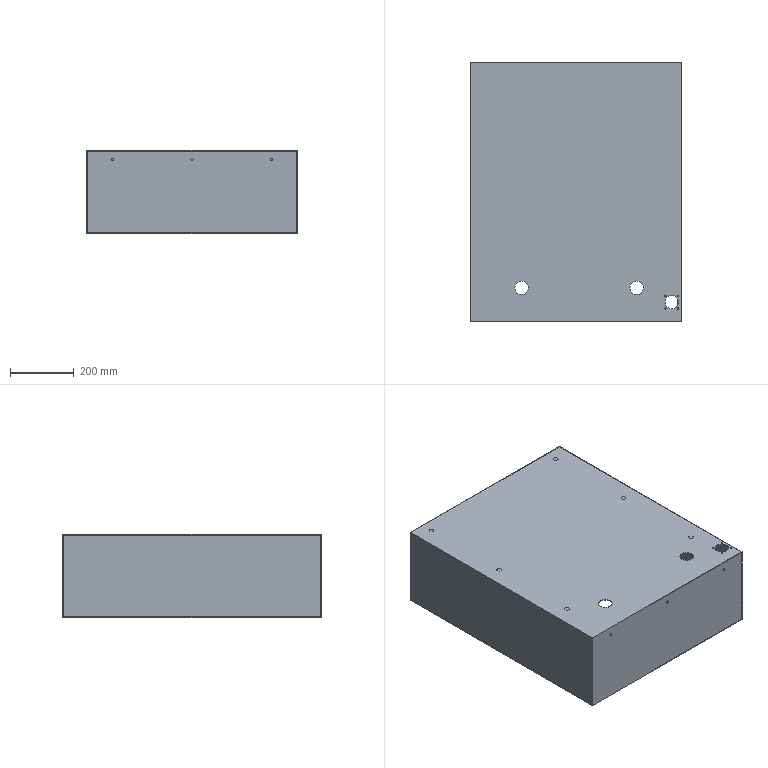Component | SolidWorks | 30-01A-1_ElectricalControlBox-1_DistributionBox1-1 | 1 solid | 118 faces | volume 2643230 mm3 | cylinder 56 | plane 50 | cone 12 | commonest cylinder face diameters 8 x12 15 x12 3.9 x8 42 x8 7 x6 4.2 x6 64 x4